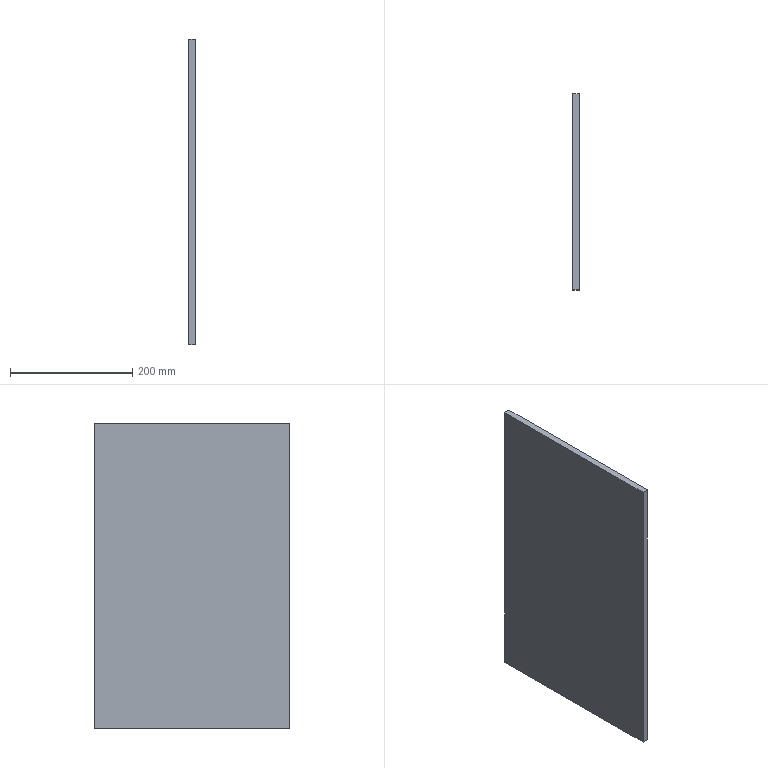Component | SolidWorks | Cover1-1 | 1 solid | 6 faces | box 10 x 320 x 500 mm | volume 1600000 mm3 | plane 6 | material Plain Carbon Steel
STEP:
#1=CARTESIAN_POINT('',(9.865,55.762,65.082));
#2=VERTEX_POINT('',#1);
#3=CARTESIAN_POINT('',(9.865,55.762,84.767));
#4=VERTEX_POINT('',#3);
#5=CARTESIAN_POINT('',(9.865,55.762,84.767));
#6=DIRECTION('',(0.,-0.,1.));
#7=VECTOR('',#6,39.37);
#8=LINE('',#5,#7);
#9=EDGE_CURVE('',#2,#4,#8,.T.);
#10=ORIENTED_EDGE('',*,*,#9,.F.);
#11=CARTESIAN_POINT('',(9.472,55.762,65.082));
#12=VERTEX_POINT('',#11);
#13=CARTESIAN_POINT('',(9.472,55.762,65.082));
#14=DIRECTION('',(1.,0.,0.));
#15=VECTOR('',#14,39.37);
#16=LINE('',#13,#15);
#17=EDGE_CURVE('',#12,#2,#16,.T.);
#18=ORIENTED_EDGE('',*,*,#17,.F.);
#19=CARTESIAN_POINT('',(9.472,55.762,84.767));
#20=VERTEX_POINT('',#19);
#21=CARTESIAN_POINT('',(9.472,55.762,84.767));
#22=DIRECTION('',(0.,-0.,1.));
#23=VECTOR('',#22,39.37);
#24=LINE('',#21,#23);
#25=EDGE_CURVE('',#12,#20,#24,.T.);
#26=ORIENTED_EDGE('',*,*,#25,.T.);
#27=CARTESIAN_POINT('',(9.472,55.762,84.767));
#28=DIRECTION('',(1.,0.,0.));
#29=VECTOR('',#28,39.37);
#30=LINE('',#27,#29);
#31=EDGE_CURVE('',#20,#4,#30,.T.);
#32=ORIENTED_EDGE('',*,*,#31,.T.);
#33=EDGE_LOOP('',(#10,#18,#26,#32));
#34=FACE_OUTER_BOUND('',#33,.T.);
#35=CARTESIAN_POINT('',(9.472,55.762,84.767));
#36=DIRECTION('',(-0.,1.,0.));
#37=DIRECTION('',(0.,-0.,1.));
#38=AXIS2_PLACEMENT_3D('',#35,#36,#37);
#39=PLANE('',#38);
#40=ADVANCED_FACE('',(#34),#39,.T.);
#41=CARTESIAN_POINT('',(9.865,43.163,65.082));
#42=VERTEX_POINT('',#41);
#43=CARTESIAN_POINT('',(9.865,43.163,65.082));
#44=DIRECTION('',(-0.,1.,0.));
#45=VECTOR('',#44,39.37);
#46=LINE('',#43,#45);
#47=EDGE_CURVE('',#42,#2,#46,.T.);
#48=ORIENTED_EDGE('',*,*,#47,.F.);
#49=CARTESIAN_POINT('',(9.472,43.163,65.082));
#50=VERTEX_POINT('',#49);
#51=CARTESIAN_POINT('',(9.472,43.163,65.082));
#52=DIRECTION('',(1.,0.,0.));
#53=VECTOR('',#52,39.37);
#54=LINE('',#51,#53);
#55=EDGE_CURVE('',#50,#42,#54,.T.);
#56=ORIENTED_EDGE('',*,*,#55,.F.);
#57=CARTESIAN_POINT('',(9.472,43.163,65.082));
#58=DIRECTION('',(-0.,1.,0.));
#59=VECTOR('',#58,39.37);
#60=LINE('',#57,#59);
#61=EDGE_CURVE('',#50,#12,#60,.T.);
#62=ORIENTED_EDGE('',*,*,#61,.T.);
#63=ORIENTED_EDGE('',*,*,#17,.T.);
#64=EDGE_LOOP('',(#48,#56,#62,#63));
#65=FACE_OUTER_BOUND('',#64,.T.);
#66=CARTESIAN_POINT('',(9.472,43.163,65.082));
#67=DIRECTION('',(0.,0.,-1.));
#68=DIRECTION('',(-1.,-0.,-0.));
#69=AXIS2_PLACEMENT_3D('',#66,#67,#68);
#70=PLANE('',#69);
#71=ADVANCED_FACE('',(#65),#70,.T.);
#72=CARTESIAN_POINT('',(9.865,43.163,84.767));
#73=VERTEX_POINT('',#72);
#74=CARTESIAN_POINT('',(9.865,43.163,84.767));
#75=DIRECTION('',(-0.,0.,-1.));
#76=VECTOR('',#75,39.37);
#77=LINE('',#74,#76);
#78=EDGE_CURVE('',#73,#42,#77,.T.);
#79=ORIENTED_EDGE('',*,*,#78,.F.);
#80=CARTESIAN_POINT('',(9.472,43.163,84.767));
#81=VERTEX_POINT('',#80);
#82=CARTESIAN_POINT('',(9.472,43.163,84.767));
#83=DIRECTION('',(1.,0.,0.));
#84=VECTOR('',#83,39.37);
#85=LINE('',#82,#84);
#86=EDGE_CURVE('',#81,#73,#85,.T.);
#87=ORIENTED_EDGE('',*,*,#86,.F.);
#88=CARTESIAN_POINT('',(9.472,43.163,84.767));
#89=DIRECTION('',(-0.,0.,-1.));
#90=VECTOR('',#89,39.37);
#91=LINE('',#88,#90);
#92=EDGE_CURVE('',#81,#50,#91,.T.);
#93=ORIENTED_EDGE('',*,*,#92,.T.);
#94=ORIENTED_EDGE('',*,*,#55,.T.);
#95=EDGE_LOOP('',(#79,#87,#93,#94));
#96=FACE_OUTER_BOUND('',#95,.T.);
#97=CARTESIAN_POINT('',(9.472,43.163,84.767));
#98=DIRECTION('',(0.,-1.,-0.));
#99=DIRECTION('',(-0.,0.,-1.));
#100=AXIS2_PLACEMENT_3D('',#97,#98,#99);
#101=PLANE('',#100);
#102=ADVANCED_FACE('',(#96),#101,.T.);
#103=CARTESIAN_POINT('',(9.865,43.163,84.767));
#104=DIRECTION('',(0.,-1.,-0.));
#105=VECTOR('',#104,39.37);
#106=LINE('',#103,#105);
#107=EDGE_CURVE('',#4,#73,#106,.T.);
#108=ORIENTED_EDGE('',*,*,#107,.F.);
#109=ORIENTED_EDGE('',*,*,#31,.F.);
#110=CARTESIAN_POINT('',(9.472,43.163,84.767));
#111=DIRECTION('',(0.,-1.,-0.));
#112=VECTOR('',#111,39.37);
#113=LINE('',#110,#112);
#114=EDGE_CURVE('',#20,#81,#113,.T.);
#115=ORIENTED_EDGE('',*,*,#114,.T.);
#116=ORIENTED_EDGE('',*,*,#86,.T.);
#117=EDGE_LOOP('',(#108,#109,#115,#116));
#118=FACE_OUTER_BOUND('',#117,.T.);
#119=CARTESIAN_POINT('',(9.472,43.163,84.767));
#120=DIRECTION('',(-0.,-0.,1.));
#121=DIRECTION('',(1.,0.,0.));
#122=AXIS2_PLACEMENT_3D('',#119,#120,#121);
#123=PLANE('',#122);
#124=ADVANCED_FACE('',(#118),#123,.T.);
#125=ORIENTED_EDGE('',*,*,#25,.F.);
#126=ORIENTED_EDGE('',*,*,#61,.F.);
#127=ORIENTED_EDGE('',*,*,#92,.F.);
#128=ORIENTED_EDGE('',*,*,#114,.F.);
#129=EDGE_LOOP('',(#125,#126,#127,#128));
#130=FACE_OUTER_BOUND('',#129,.T.);
#131=CARTESIAN_POINT('',(9.472,49.463,74.925));
#132=DIRECTION('',(1.,0.,0.));
#133=DIRECTION('',(-0.,1.,0.));
#134=AXIS2_PLACEMENT_3D('',#131,#132,#133);
#135=PLANE('',#134);
#136=ADVANCED_FACE('',(#130),#135,.F.);
#137=ORIENTED_EDGE('',*,*,#9,.T.);
#138=ORIENTED_EDGE('',*,*,#107,.T.);
#139=ORIENTED_EDGE('',*,*,#78,.T.);
#140=ORIENTED_EDGE('',*,*,#47,.T.);
#141=EDGE_LOOP('',(#137,#138,#139,#140));
#142=FACE_OUTER_BOUND('',#141,.T.);
#143=CARTESIAN_POINT('',(9.865,49.463,74.925));
#144=DIRECTION('',(1.,0.,0.));
#145=DIRECTION('',(-0.,1.,0.));
#146=AXIS2_PLACEMENT_3D('',#143,#144,#145);
#147=PLANE('',#146);
#148=ADVANCED_FACE('',(#142),#147,.T.);
#149=CLOSED_SHELL('',(#40,#71,#102,#124,#136,#148));
#150=MANIFOLD_SOLID_BREP('',#149);
#151=CARTESIAN_POINT('',(0.,0.,0.));
#152=DIRECTION('',(0.,0.,1.));
#153=DIRECTION('',(1.,0.,0.));
#154=AXIS2_PLACEMENT_3D('',#151,#152,#153);
#155=(LENGTH_UNIT()NAMED_UNIT(*)SI_UNIT($,.METRE.));
#156=LENGTH_MEASURE_WITH_UNIT(LENGTH_MEASURE(0.0254),#155);
#157=DIMENSIONAL_EXPONENTS(1.,0.,0.,0.,0.,0.,0.);
#158=(CONVERSION_BASED_UNIT('',#156)LENGTH_UNIT()NAMED_UNIT(#157));
#159=UNCERTAINTY_MEASURE_WITH_UNIT(LENGTH_MEASURE(0.00001),#158,'','');
#160=(NAMED_UNIT(*)PLANE_ANGLE_UNIT()SI_UNIT($,.RADIAN.));
#161=(NAMED_UNIT(*)SI_UNIT($,.STERADIAN.)SOLID_ANGLE_UNIT());
#162=(GEOMETRIC_REPRESENTATION_CONTEXT(3)GLOBAL_UNCERTAINTY_ASSIGNED_CONTEXT((#159))GLOBAL_UNIT_ASSIGNED_CONTEXT((#158,#160,#161))REPRESENTATION_CONTEXT('',''));
#163=ADVANCED_BREP_SHAPE_REPRESENTATION('',(#150,#154),#162);
#164=COLOUR_RGB('',0.7922,0.8196,0.9333);
#165=FILL_AREA_STYLE_COLOUR('',#164);
#166=FILL_AREA_STYLE('',(#165));
#167=SURFACE_STYLE_FILL_AREA(#166);
#168=SURFACE_SIDE_STYLE('',(#167));
#169=SURFACE_STYLE_USAGE(.BOTH.,#168);
#170=PRESENTATION_STYLE_ASSIGNMENT((#169));
#171=STYLED_ITEM('',(#170),#150);
#172=PRESENTATION_LAYER_ASSIGNMENT('','',(#171));
#173=(LENGTH_UNIT()NAMED_UNIT(*)SI_UNIT($,.METRE.));
#174=LENGTH_MEASURE_WITH_UNIT(LENGTH_MEASURE(0.0254),#173);
#175=DIMENSIONAL_EXPONENTS(1.,0.,0.,0.,0.,0.,0.);
#176=(CONVERSION_BASED_UNIT('',#174)LENGTH_UNIT()NAMED_UNIT(#175));
#177=UNCERTAINTY_MEASURE_WITH_UNIT(LENGTH_MEASURE(0.00001),#176,'','');
#178=(NAMED_UNIT(*)PLANE_ANGLE_UNIT()SI_UNIT($,.RADIAN.));
#179=(NAMED_UNIT(*)SI_UNIT($,.STERADIAN.)SOLID_ANGLE_UNIT());
#180=(GEOMETRIC_REPRESENTATION_CONTEXT(3)GLOBAL_UNCERTAINTY_ASSIGNED_CONTEXT((#177))GLOBAL_UNIT_ASSIGNED_CONTEXT((#176,#178,#179))REPRESENTATION_CONTEXT('',''));
#181=MECHANICAL_DESIGN_GEOMETRIC_PRESENTATION_REPRESENTATION('',(#171),#180);